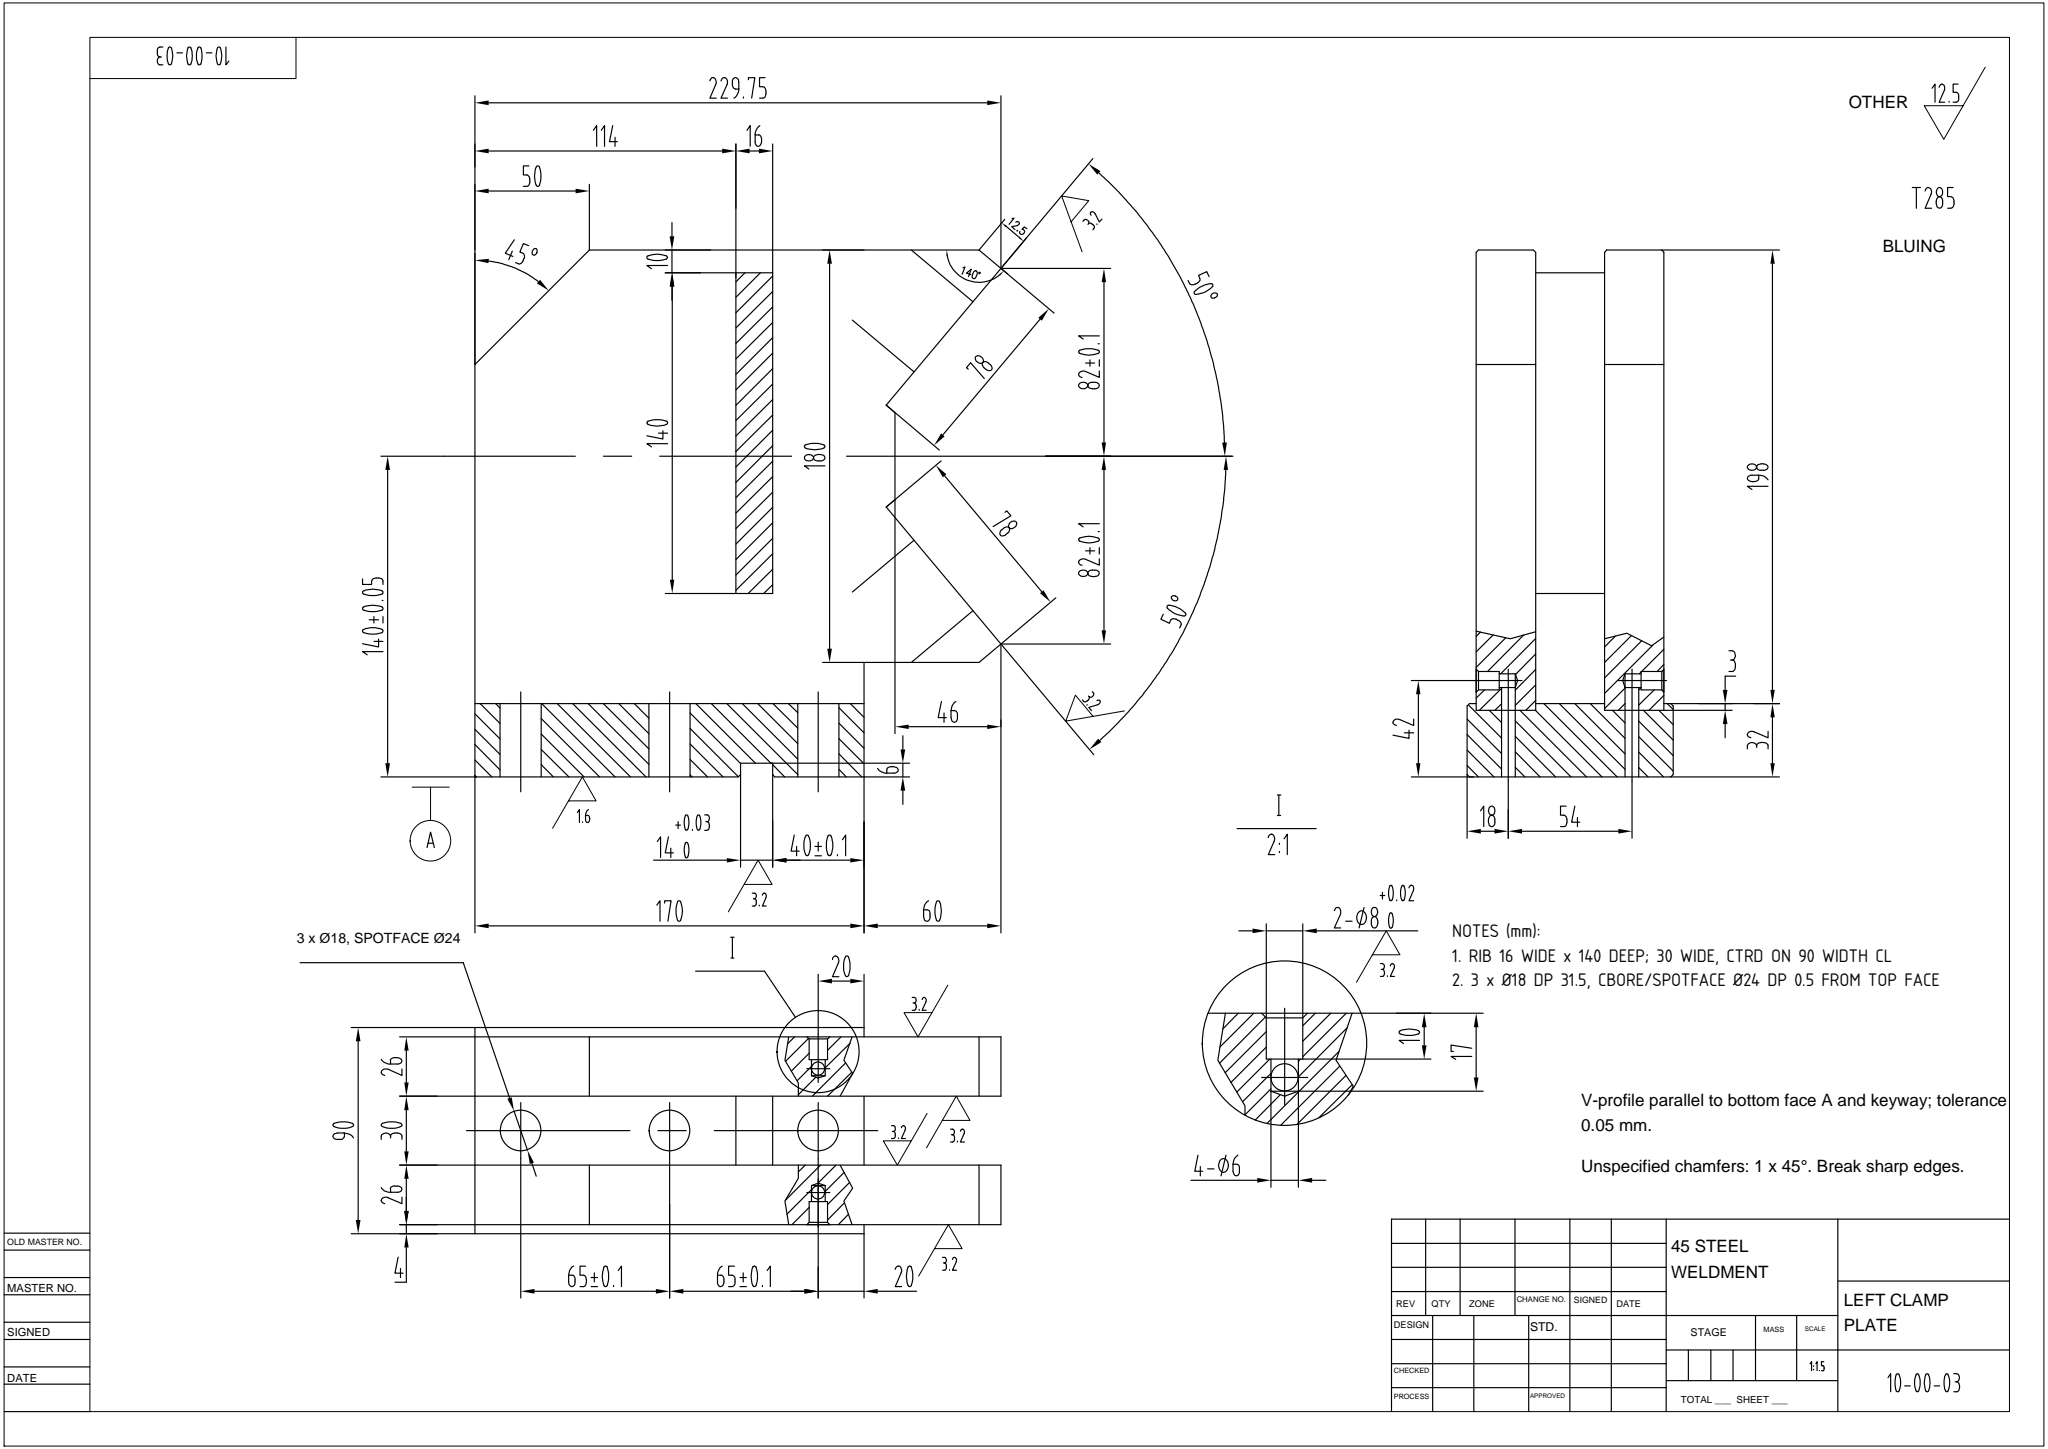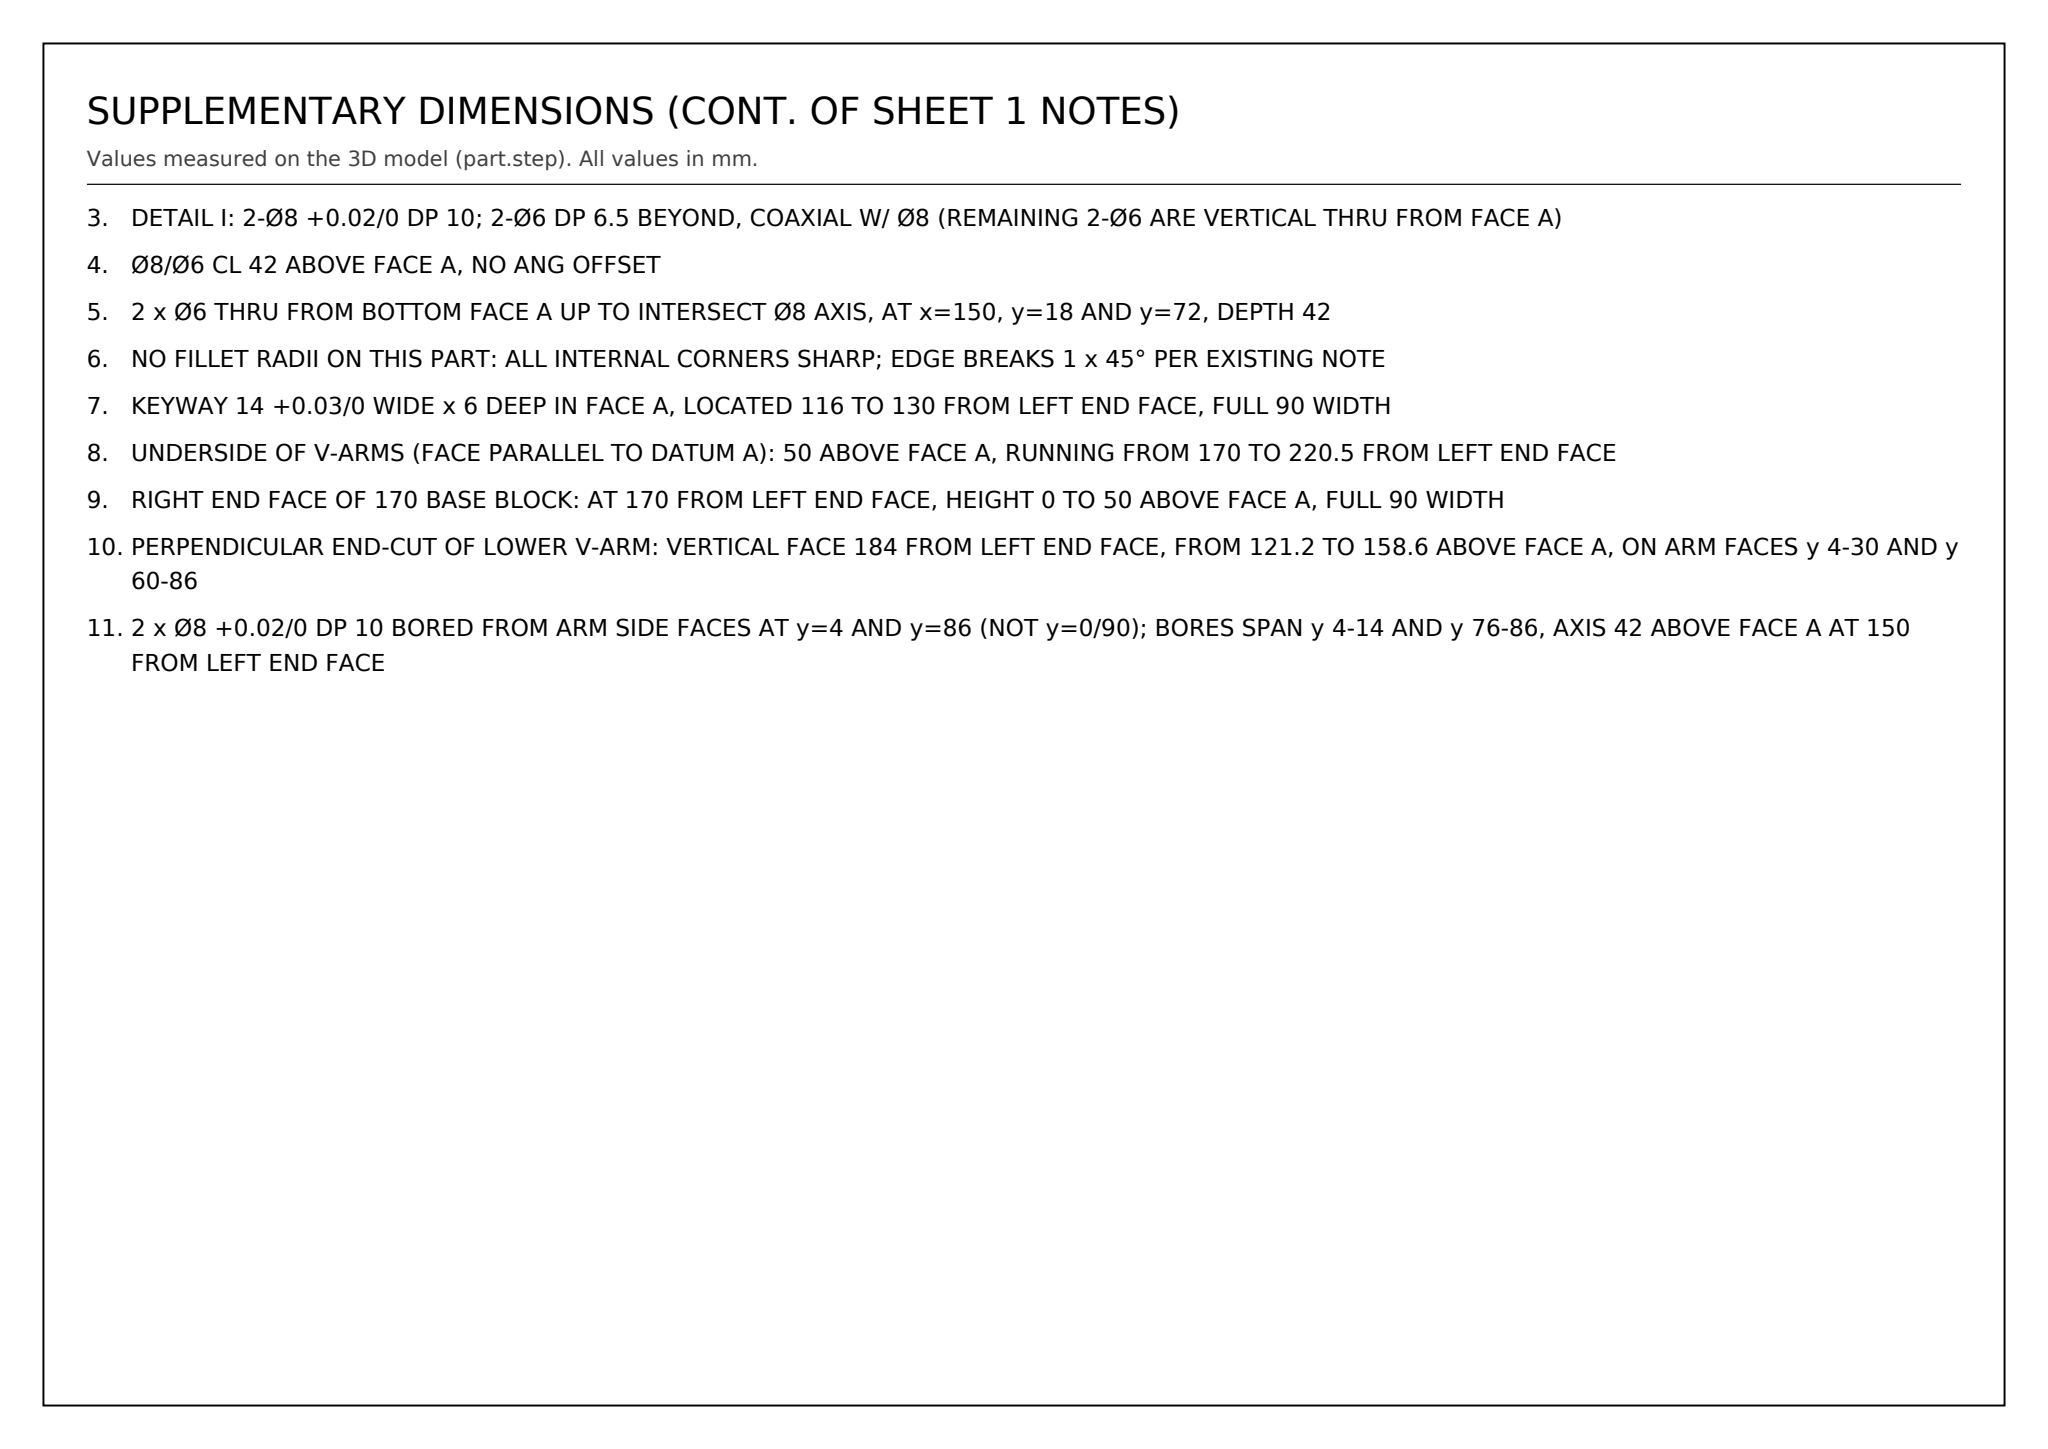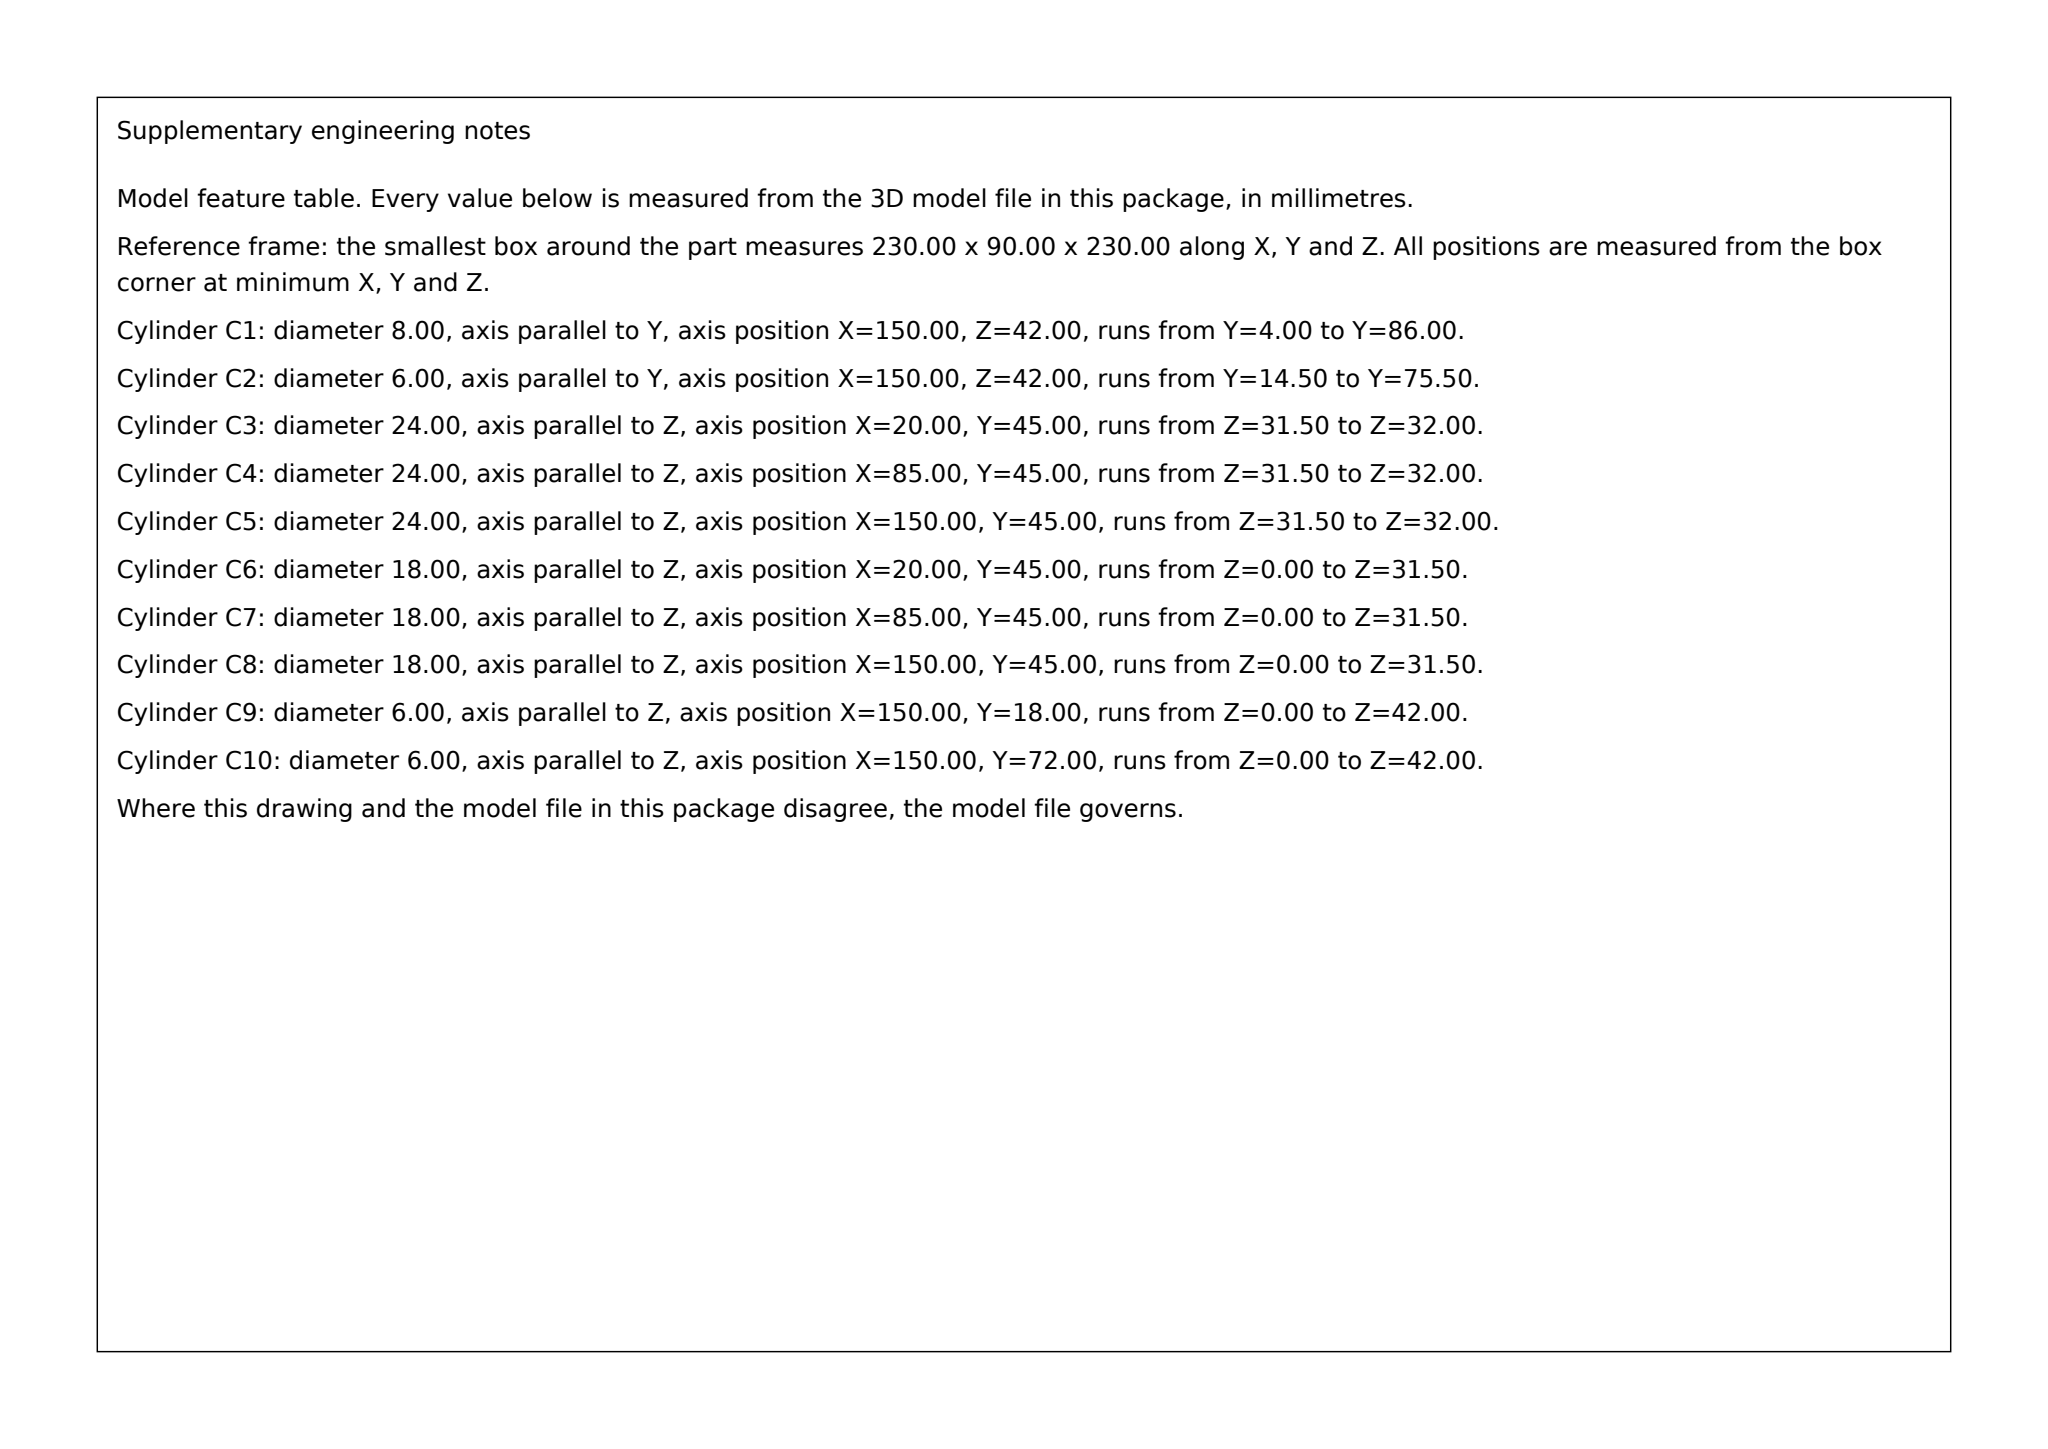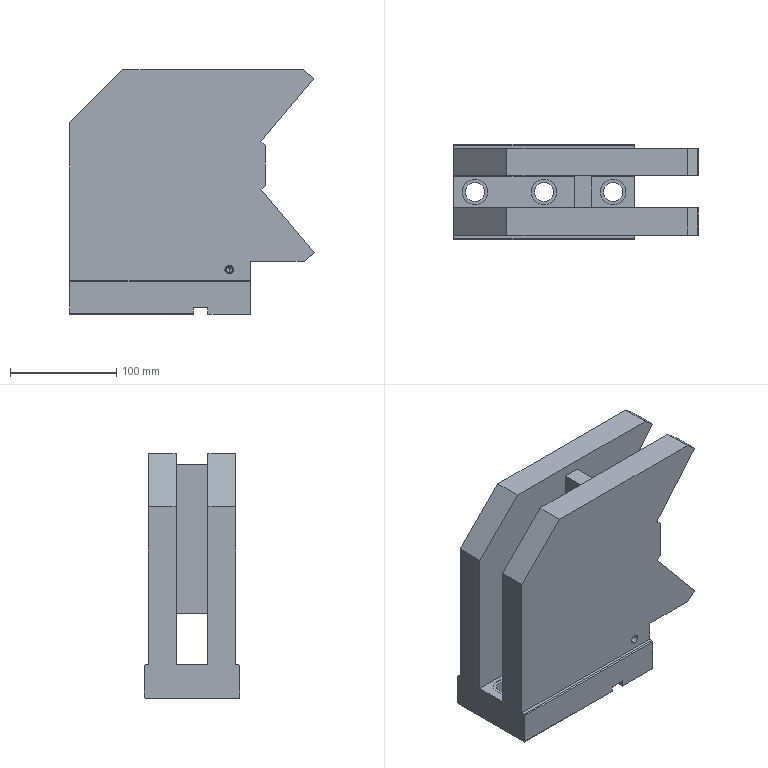Part | SolidWorks | mm | 1 solid | 82 faces | box 230 x 90 x 230 mm | volume 2499743 mm3 | plane 50 | cylinder 24 | cone 8 | commonest cylinder face diameters 6 x8 24 x6 18 x6 8 x4
Drawing notes:
RIB 16 WIDE x 140 DEEP; 30 WIDE, CTRD ON 90 WIDTH CL | from the solid: x-planes 114 & 130 (16 wide); y-planes 30 & 60 (30 wide, ctr y=45=90/2); z 80 to 220 = 140 deep
3 x Ø18 DP 31.5, CBORE/SPOTFACE Ø24 DP 0.5 FROM TOP FACE | from the solid: dia18 axis z len31.5 at x=20,85,150 y=45; dia24 axis z len0.5 same axes
DETAIL I: 2-Ø8 +0.02/0 DP 10; 2-Ø6 DP 6.5 BEYOND, COAXIAL W/ Ø8 (REMAINING 2-Ø6 ARE VERTICAL THRU FROM FACE A) | from the solid: Only two Ø6 bores are coaxial with the Ø8 axis: y-axis Ø6 at [150,-,42] from y 14.5 to 21.0 and from y 69.0 to 75.5 (6.5 deep each). The other two Ø6 are z-axis holes at [150,18] and [150,72] running z 0 to 42, i.e. not coaxial with Ø8.
Ø8/Ø6 CL 42 ABOVE FACE A, NO ANG OFFSET | from the solid: dia6 & dia8 axis y share pos [150,-,42]; z=42 above bottom face z=0
2 x Ø6 THRU FROM BOTTOM FACE A UP TO INTERSECT Ø8 AXIS, AT x=150, y=18 AND y=72, DEPTH 42 | from the solid: cylinders Ø6 z-axis at (150,18) and (150,72) from 0 to 42
NO FILLET RADII ON THIS PART: ALL INTERNAL CORNERS SHARP; EDGE BREAKS 1 x 45° PER EXISTING NOTE | from the solid: tori[minor_r,major_r] list is empty (no blend/fillet faces in model)
KEYWAY 14 +0.03/0 WIDE x 6 DEEP IN FACE A, LOCATED 116 TO 130 FROM LEFT END FACE, FULL 90 WIDTH | from the solid: axis_planes x=116 and x=130 extent y[0,90] z[0,6]; z=6 extent x[116,130] y[0,90]
UNDERSIDE OF V-ARMS (FACE PARALLEL TO DATUM A): 50 ABOVE FACE A, RUNNING FROM 170 TO 220.5 FROM LEFT END FACE | from the solid: axis_planes z=50, extent x[170.0,220.5], y[4,30] and y[60,86]
RIGHT END FACE OF 170 BASE BLOCK: AT 170 FROM LEFT END FACE, HEIGHT 0 TO 50 ABOVE FACE A, FULL 90 WIDTH | from the solid: axis_planes x=170, extent y[0,90], z[0,50], area 3814
PERPENDICULAR END-CUT OF LOWER V-ARM: VERTICAL FACE 184 FROM LEFT END FACE, FROM 121.2 TO 158.6 ABOVE FACE A, ON ARM FACES y 4-30 AND y 60-86 | from the solid: axis_planes x=184, extent z[121.2,158.6], y[4,30] and y[60,86]
2 x Ø8 +0.02/0 DP 10 BORED FROM ARM SIDE FACES AT y=4 AND y=86 (NOT y=0/90); BORES SPAN y 4-14 AND y 76-86, AXIS 42 ABOVE FACE A AT 150 FROM LEFT END FACE | from the solid: cylinders Ø8 axis y at [150,-,42], from 4.0 to 14.0 and from 76.0 to 86.0